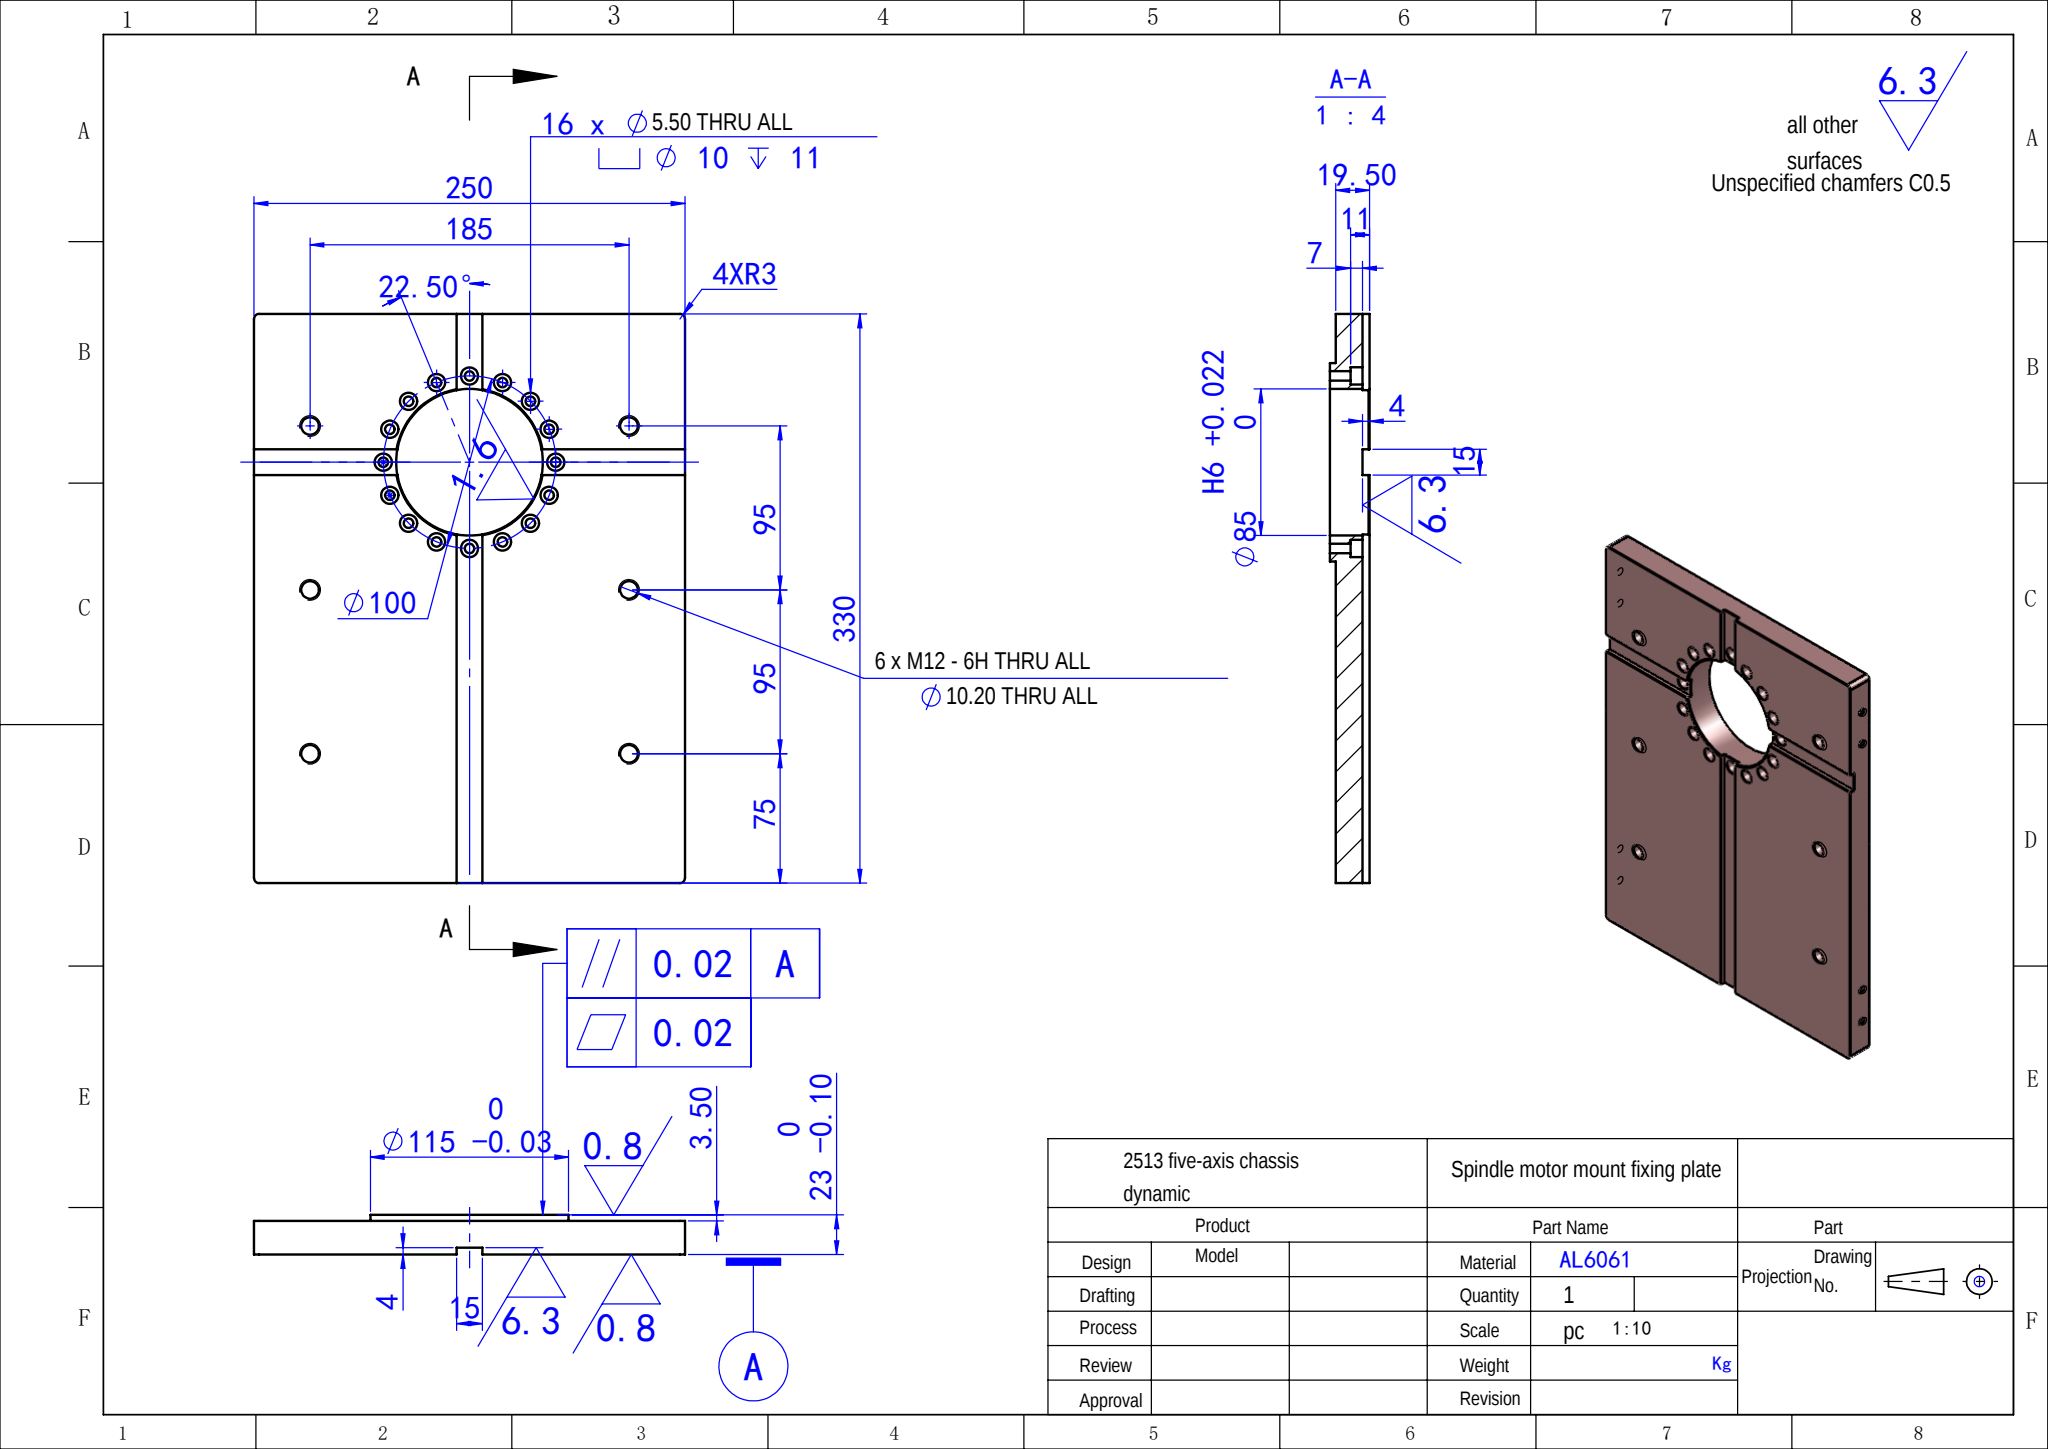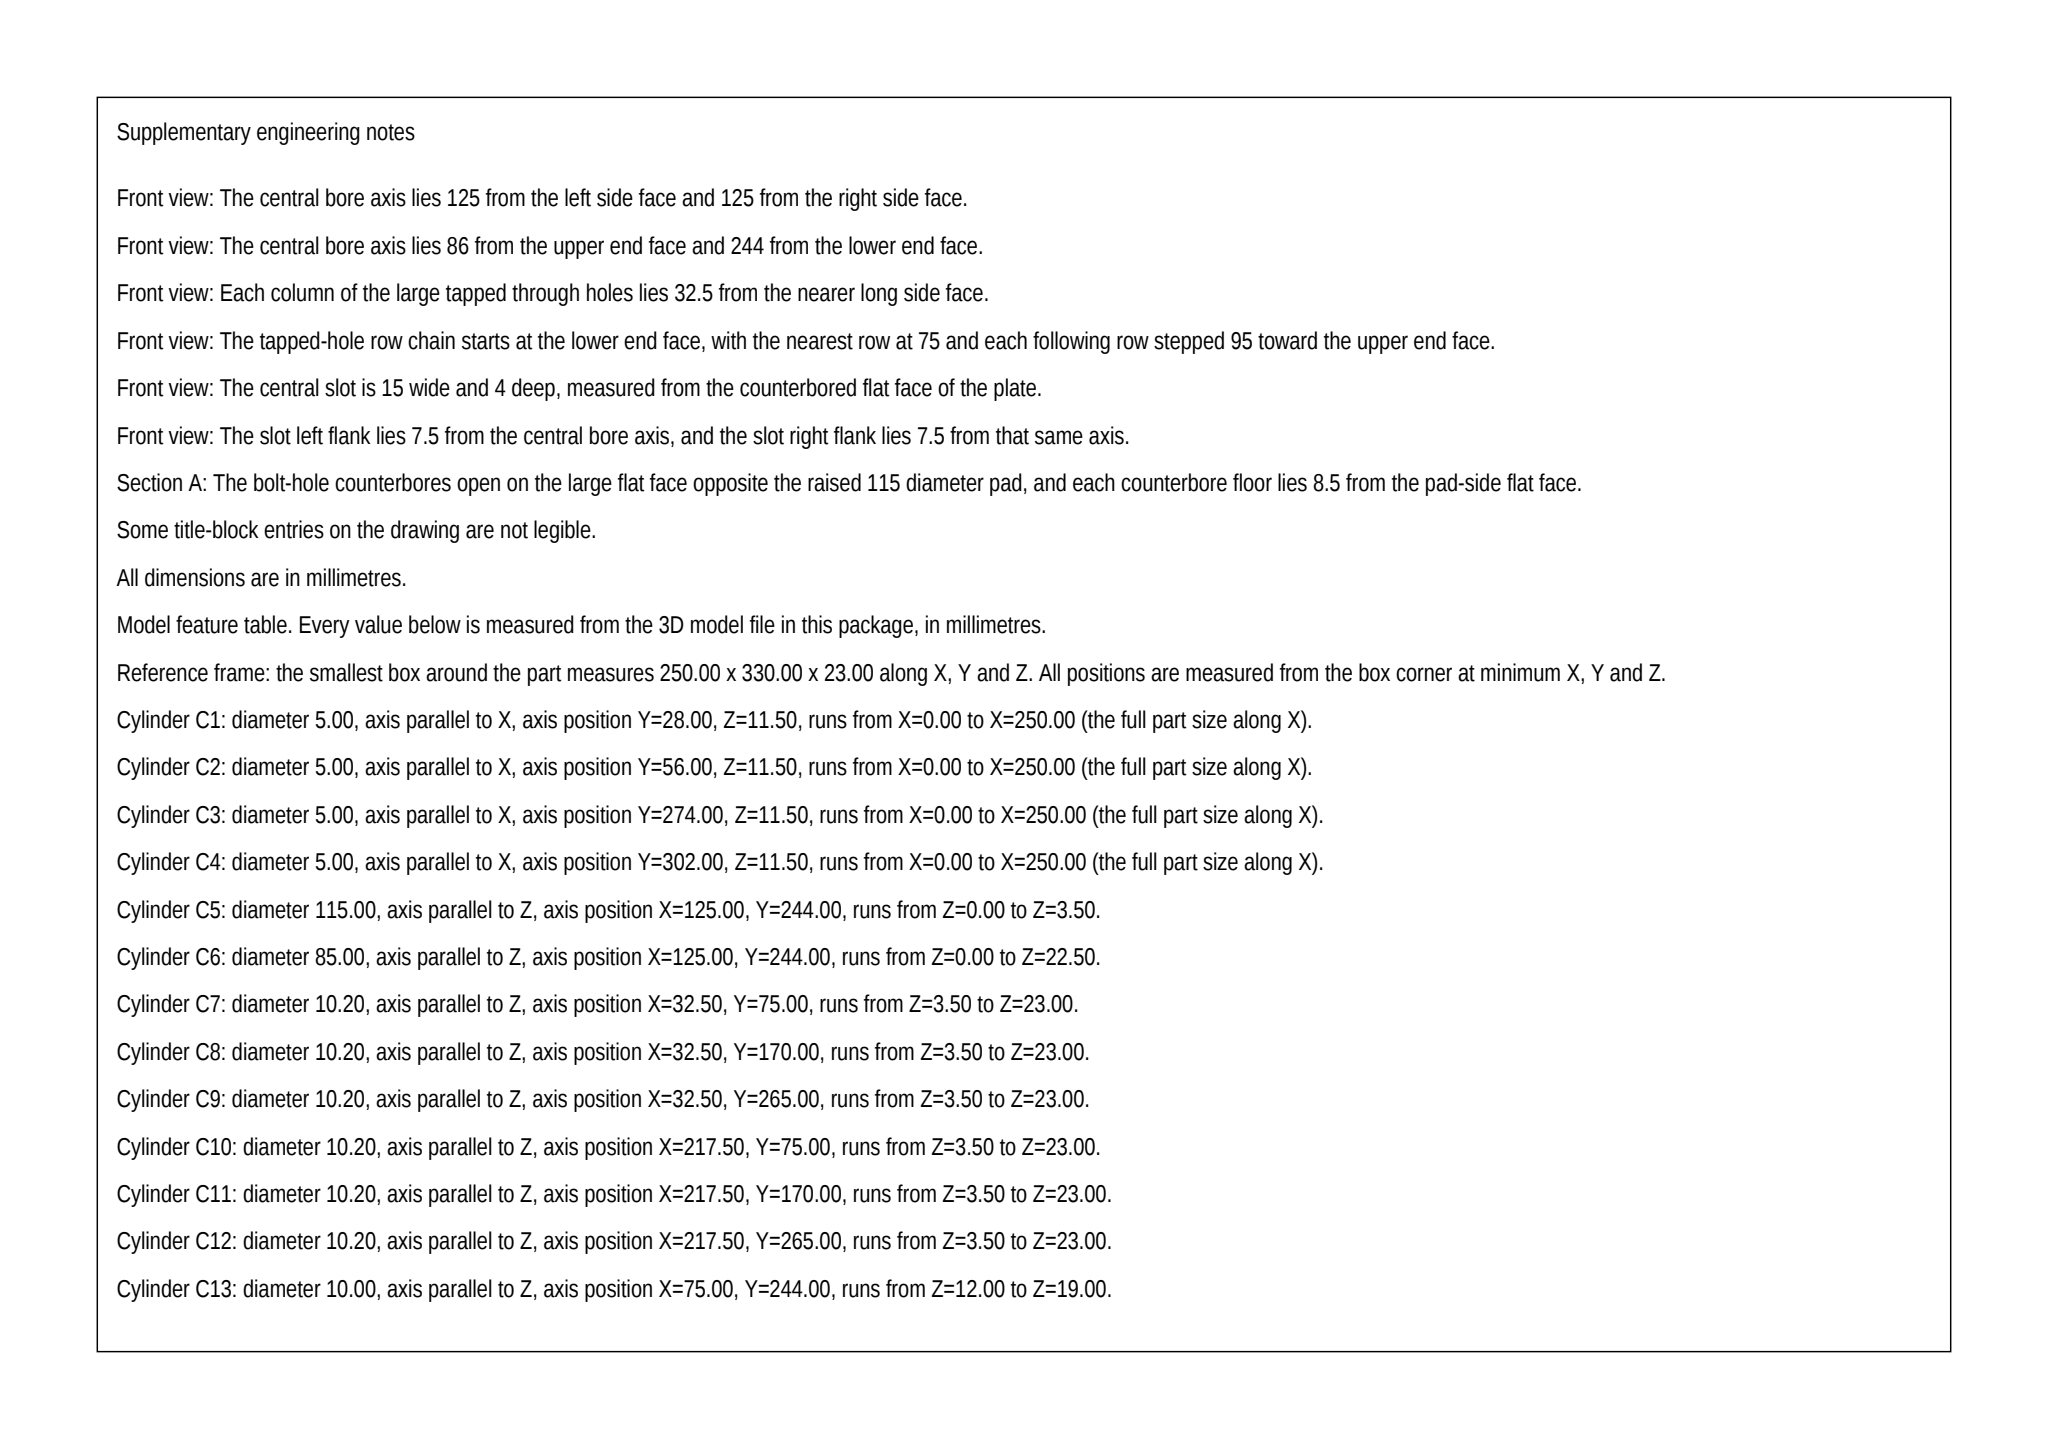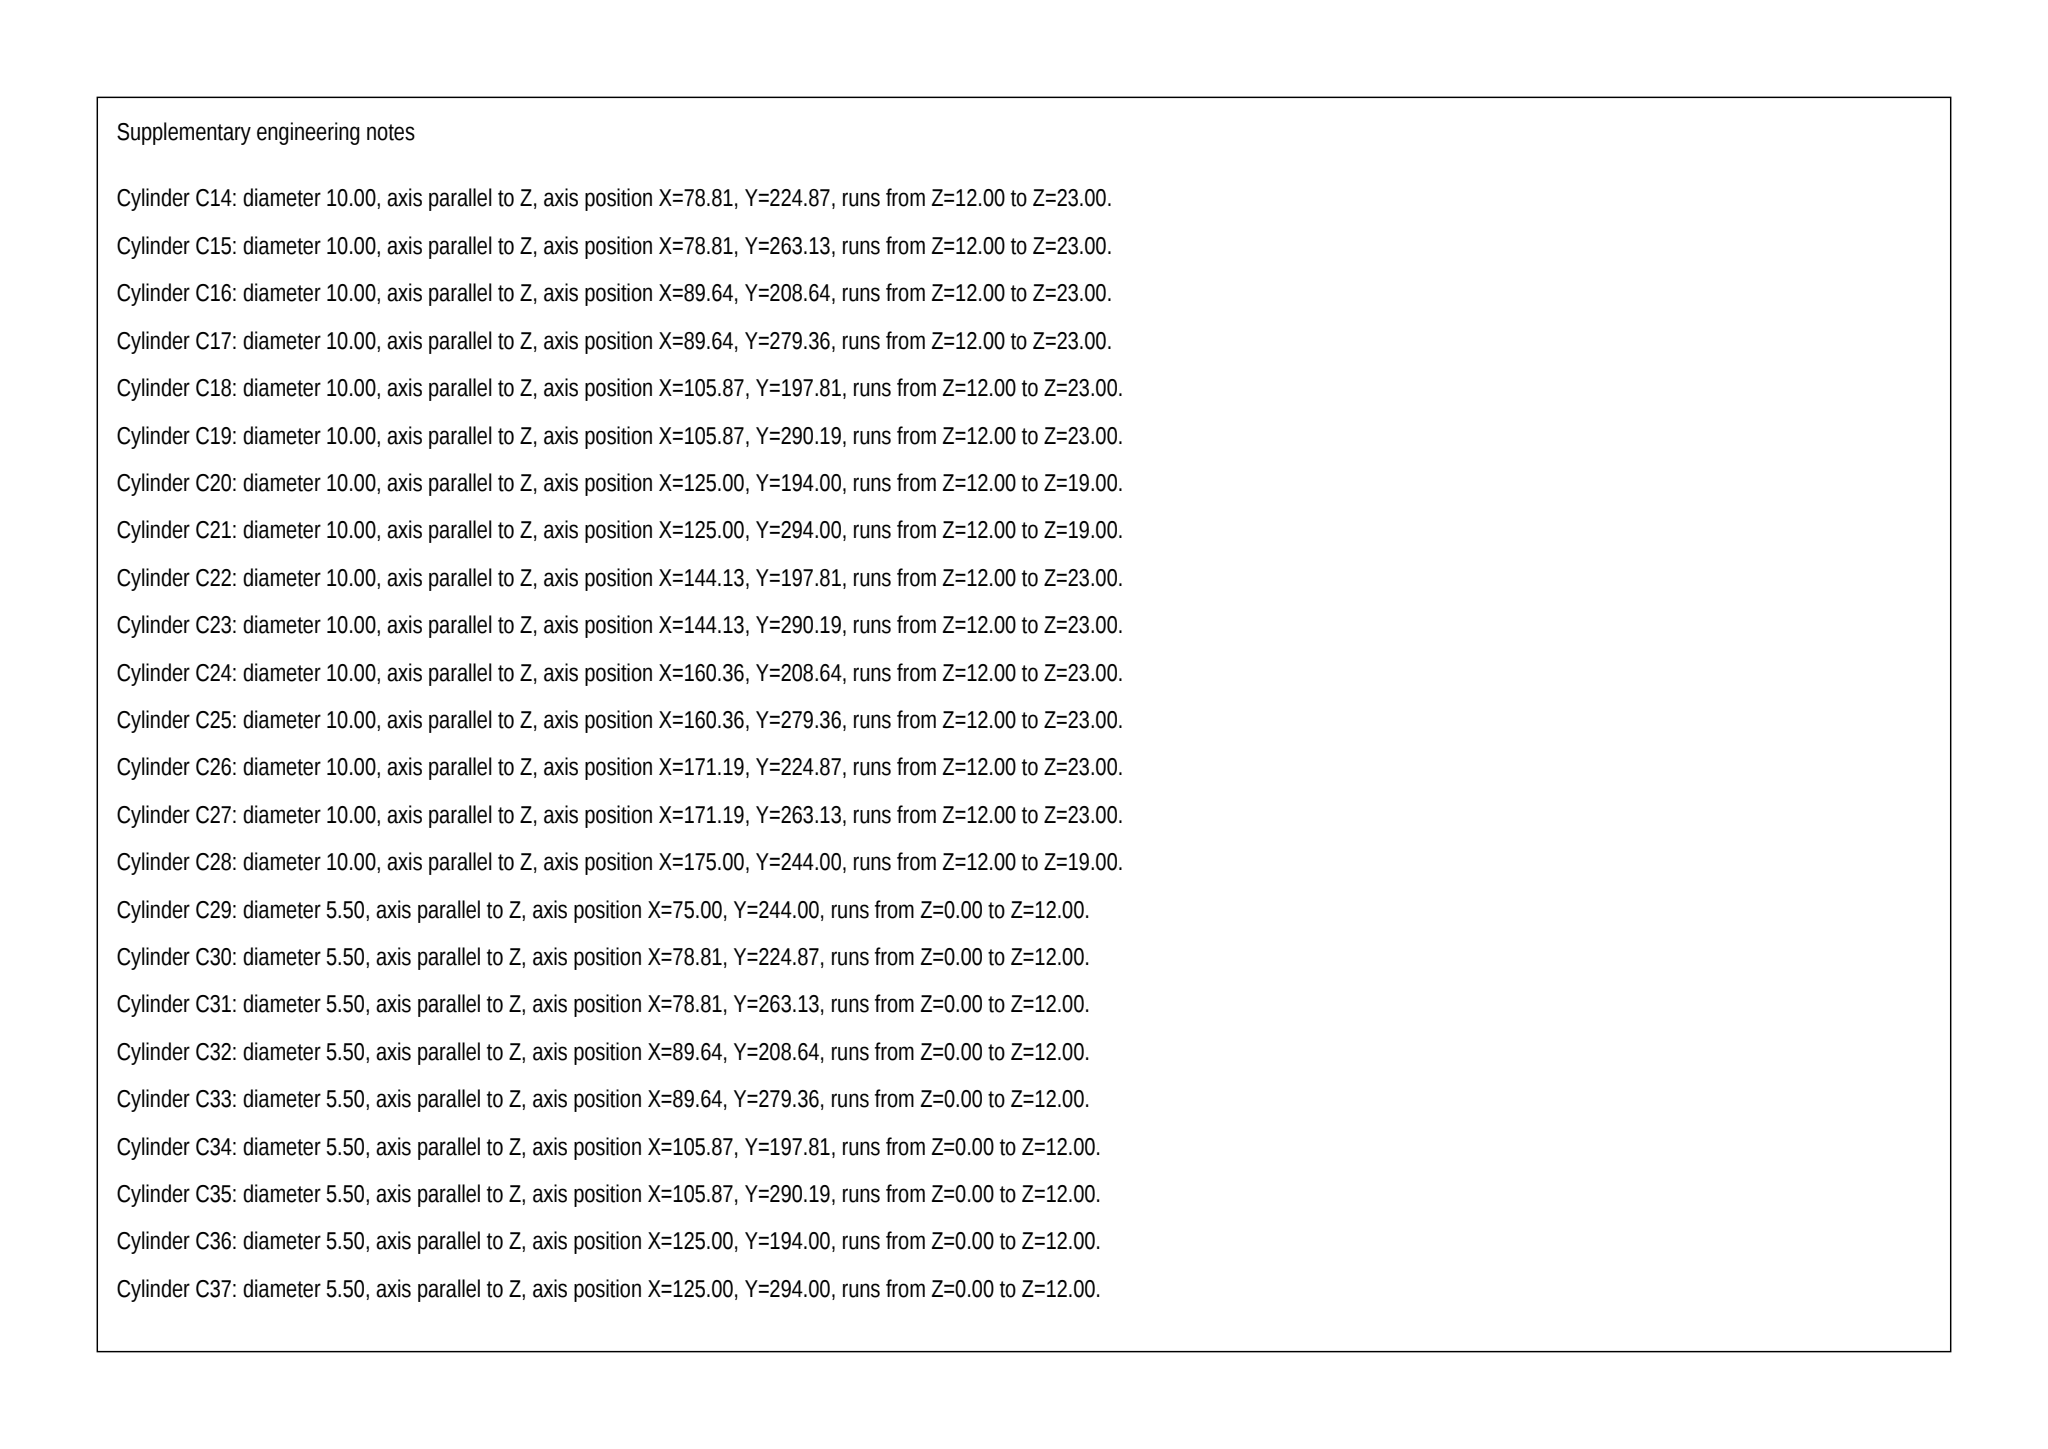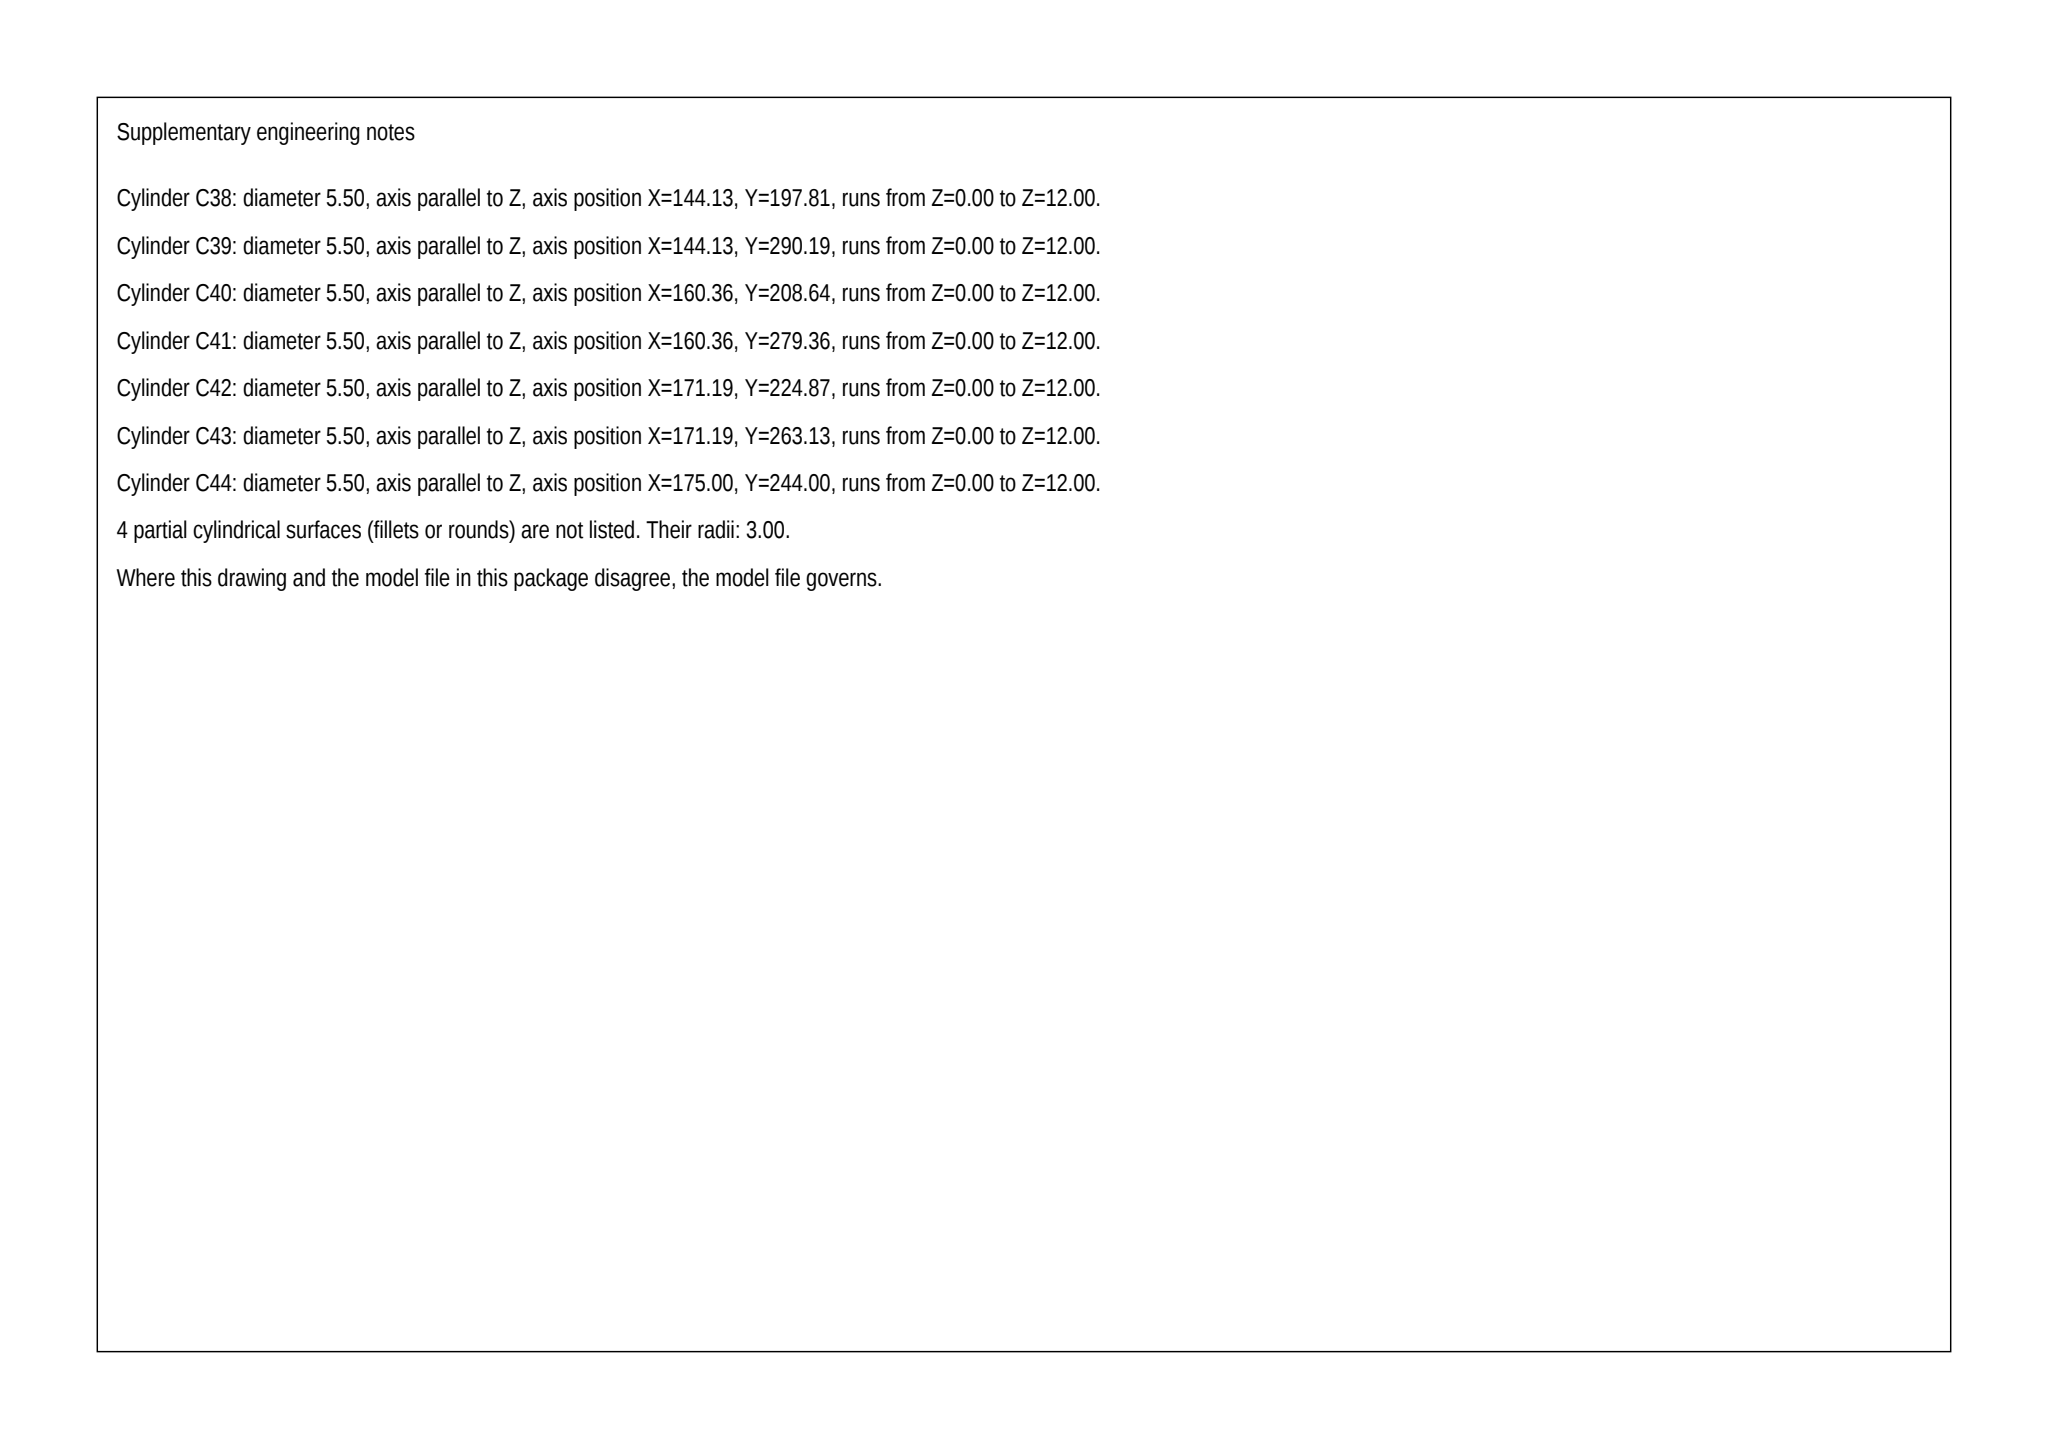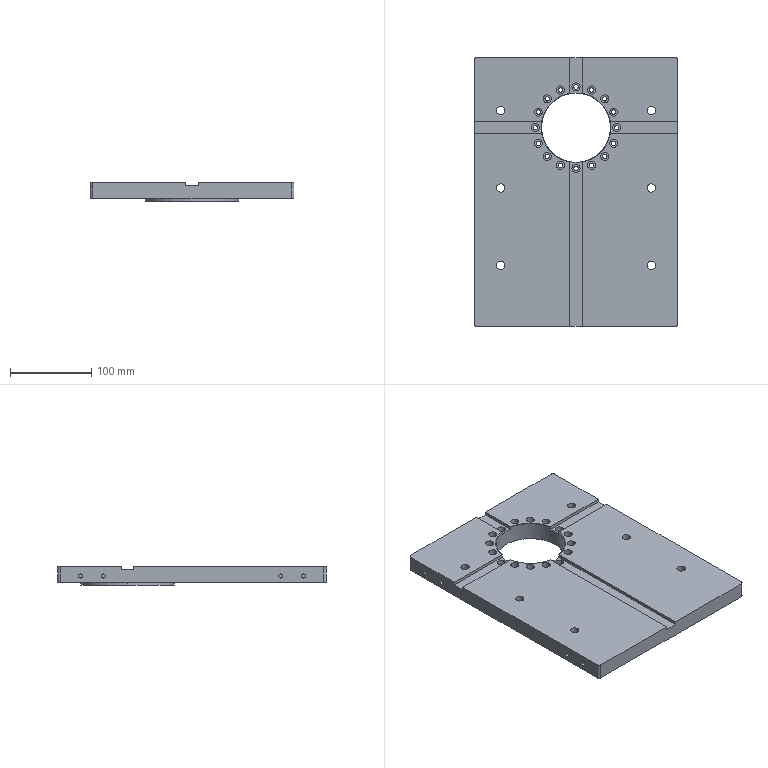Part | SolidWorks | mm | material AL6061 | 1 solid | 150 faces | box 250 x 330 x 23 mm | volume 1460716 mm3 | cylinder 100 | plane 46 | cone 4 | commonest cylinder face diameters 10 x32 5.5 x32 5 x16 10.2 x12 6 x4 115 x2 85 x2
Drawing notes:
8X Ø5 DP 15 SIDE HOLES: AXES 11.5 FROM BACK FACE (CL OF 23 THK) | from the solid: Ø5 x-axis cylinders at z=11.5, plate thk 23 (z 0..23); 11.5 = mid-thickness
build123d program:
from build123d import *
from build123d.topology import SkipClean

# Parameters (mm, degrees)
SKETCH1_W                                         = 250
SKETCH1_H                                         = 330
SKETCH1_R                                         = 42.5
BOSS_EXTRUDE1_DEPTH                               = 19.5
BOSS_EXTRUDE2_START                               = 3.5
SKETCH8_R                                         = 57.5
SKETCH8_R_2                                       = 42.5
BOSS_EXTRUDE2_DEPTH                               = 3.5
HOLE_SIZE_ACCORDING_TO_TYPE_OF_HEXAGO_D           = 5.5
HOLE_SIZE_ACCORDING_TO_TYPE_OF_HEXAGO_CBORE_D     = 10
HOLE_SIZE_ACCORDING_TO_TYPE_OF_HEXAGO_CBORE_DEPTH = 11
CIRPATTERN2_COUNT                                 = 16
M12_TAPPED_HOLE1_D                                = 10.2
FILLET1_R                                         = 3
CHAMFER1_SIZE                                     = 0.5
SKETCH17_W                                        = 15
SKETCH17_H                                        = 330
CUT_EXTRUDE1_DEPTH                                = 4
CUT_EXTRUDE2_REACH                                = 277.118
M6_TAPPED_HOLE1_D                                 = 5
M6_TAPPED_HOLE1_DEPTH                             = 15
MIRROR4_COPY_1_D                                  = 5
MIRROR4_COPY_1_DEPTH                              = 15


with BuildPart() as part:
    # Sketch1 → Boss-Extrude1 (new body)
    with BuildSketch(Plane.XY):
        with Locations((0, -79)):
            Rectangle(SKETCH1_W, SKETCH1_H)
        Circle(SKETCH1_R, mode=Mode.SUBTRACT)
    extrude(amount=BOSS_EXTRUDE1_DEPTH)

    # Sketch8 → Boss-Extrude2 (add)
    with SkipClean():  # the faces are left unmerged after this step: merging them gives an invalid solid
        with BuildSketch(Plane(origin=(0, 0, 0), x_dir=(-1, 0, 0), z_dir=(0, 0, -1)).offset(BOSS_EXTRUDE2_START)):
            with Locations(Location((0, 0, 0), (0, 0, 180))):
                Circle(SKETCH8_R)
            Circle(SKETCH8_R_2, mode=Mode.SUBTRACT)
        extrude(amount=-BOSS_EXTRUDE2_DEPTH)

    # Hole Size _ according to_ type of Hexago (through all)
    with Locations(Plane.XY.offset(19.5)):
        with Locations((50, 0)):
            hole_size_according_to_type_of_hexago = CounterBoreHole(HOLE_SIZE_ACCORDING_TO_TYPE_OF_HEXAGO_D / 2, HOLE_SIZE_ACCORDING_TO_TYPE_OF_HEXAGO_CBORE_D / 2, HOLE_SIZE_ACCORDING_TO_TYPE_OF_HEXAGO_CBORE_DEPTH)

    # CirPattern2: Hole Size _ according to_ type of Hexago ×16 about axis
    with SkipClean():  # the faces are left unmerged after this step: merging them gives an invalid solid
        cirpattern2_axis = Axis((0, 0, 0), (0, 0, 1))
        for i in range(1, CIRPATTERN2_COUNT):
            add(hole_size_according_to_type_of_hexago.rotate(cirpattern2_axis, i * 360 / CIRPATTERN2_COUNT), mode=Mode.SUBTRACT)

    # M12 Tapped Hole1 (through all)
    with Locations(Plane.XY.offset(19.5)):
        with Locations((-92.5, 21), (92.5, 21), (-92.5, -74), (92.5, -74), (-92.5, -169), (92.5, -169)):
            Hole(M12_TAPPED_HOLE1_D / 2)

    # Fillet1
    fillet1_edges = [part.edges().sort_by_distance(p)[0] for p in [
        (-125, 86, 9.75),
        (125, 86, 9.75),
        (125, -244, 9.75),
        (-125, -244, 9.75),
    ]]
    fillet(fillet1_edges, radius=FILLET1_R)

    # Chamfer1
    chamfer1_edges = [part.edges().sort_by_distance(p)[0] for p in [
        (-42.5, 0, 19.5),
    ]]
    chamfer(chamfer1_edges, length=CHAMFER1_SIZE)

    # Sketch17 → Cut-Extrude1 (cut)
    with SkipClean():  # the faces are left unmerged after this step: merging them gives an invalid solid
        with BuildSketch(Plane.XY.offset(19.5)):
            with Locations((0, -79)):
                Rectangle(SKETCH17_W, SKETCH17_H)
        extrude(amount=-CUT_EXTRUDE1_DEPTH, mode=Mode.SUBTRACT)

    # Cut-Extrude2: up to this face of the body (flat: up to its plane)
    cut_extrude2_end = Plane(part.part.faces().sort_by_distance((0, 66.062, 15.5))[0])
    # Sketch18 → Cut-Extrude2 (cut, up to the picked face)
    with BuildSketch(Plane.XY.offset(19.5), mode=Mode.PRIVATE) as cut_extrude2_sk1:
        with BuildLine():
            Line((125, 7.5), (41.833, 7.5))
            ThreePointArc((41.833, 7.5), (42.5, 0), (41.833, -7.5))
            Line((41.833, -7.5), (125, -7.5))
            Line((125, -7.5), (125, 7.5))
        make_face()
    cut_extrude2_tool1 = split(extrude(cut_extrude2_sk1.sketch, amount=-CUT_EXTRUDE2_REACH, mode=Mode.PRIVATE), bisect_by=cut_extrude2_end, keep=Keep.BOTH, mode=Mode.PRIVATE)
    cut_extrude2 = cut_extrude2_tool1.solids().sort_by(Axis((83.639, 0, 19.5), (0, 0, -1)))[0]
    add(cut_extrude2, mode=Mode.SUBTRACT)

    # Mirror2: Cut-Extrude2 across plane
    with SkipClean():  # the faces are left unmerged after this step: merging them gives an invalid solid
        add(cut_extrude2.mirror(Plane(origin=(0, 0, 0), x_dir=(0, 0, 1), z_dir=(1, 0, 0))), mode=Mode.SUBTRACT)

    # M6 Tapped Hole1
    with Locations(Plane(origin=(125, 0, 0), x_dir=(0, 0, -1), z_dir=(1, 0, 0))):
        with Locations((-8, -216), (-8, -188)):
            m6_tapped_hole1 = Hole(M6_TAPPED_HOLE1_D / 2, depth=M6_TAPPED_HOLE1_DEPTH)

    # Mirror3: M6 Tapped Hole1 across plane
    with SkipClean():  # the faces are left unmerged after this step: merging them gives an invalid solid
        add(m6_tapped_hole1.mirror(Plane(origin=(0, 0, 0), x_dir=(0, 0, 1), z_dir=(1, 0, 0))), mode=Mode.SUBTRACT)

    # Mirror4: M6 Tapped Hole1 across plane
    with SkipClean():  # the faces are left unmerged after this step: merging them gives an invalid solid
        add(m6_tapped_hole1.mirror(Plane.ZX.offset(-79)), mode=Mode.SUBTRACT)

    # Mirror4 copy 1
    with Locations(Plane(origin=(-125, -158, 0), x_dir=(0, 0, -1), z_dir=(-1, 0, 0))):
        with Locations((-8, -216), (-8, -188)):
            Hole(MIRROR4_COPY_1_D / 2, depth=MIRROR4_COPY_1_DEPTH)


solid = part.part